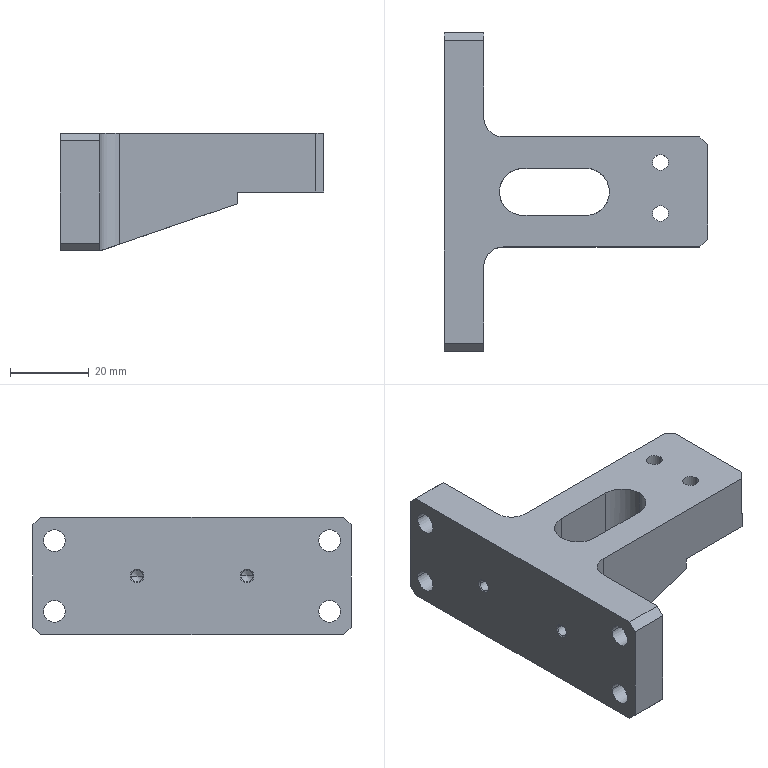Component | SolidWorks | AX.B92.SA.7371.20-2 | 1 solid | 60 faces | box 67 x 81 x 30 mm | volume 48369 mm3 | cylinder 25 | plane 23 | cone 12 | commonest cylinder face diameters 5.5 x8 4 x4 6 x4 3 x4 12 x3 10 x2 | material 6061
build123d program:
from build123d import *

# Parameters (mm, degrees)
BOSS_EXTRUDE1_DEPTH                 = 15
SKETCH2_W                           = 28
SKETCH2_H                           = 22
CUT_EXTRUDE1_DEPTH                  = 15
SKETCH3_W                           = 81
SKETCH3_H                           = 30
BOSS_EXTRUDE2_DEPTH                 = 10
FILLET2_R                           = 5
CHAMFER1_SIZE                       = 2
CUT_EXTRUDE2_DEPTH                  = 84.841
CUT_EXTRUDE3_DEPTH                  = 50
F_5_5_5_5_DIAMETER_HOLE1_D          = 5.5
SIZE_MM_DOWEL_PIN_HOLE1_D           = 3
SIZE_MM_DOWEL_PIN_HOLE1_DEPTH       = 10
SIZE_MM_DOWEL_PIN_HOLE1_CSINK_D     = 3.5
SIZE_MM_DOWEL_PIN_HOLE1_CSINK_ANGLE = 90
SIZE_MM_DOWEL_PIN_HOLE1_TIP         = 0.9013
SKETCH10_R                          = 3
CUT_EXTRUDE4_DEPTH                  = 4
M4_TAPPED_HOLE1_D                   = 4
M4_TAPPED_HOLE1_CSINK_D             = 4.05
M4_TAPPED_HOLE1_CSINK_ANGLE         = 90


with BuildPart() as part:
    # Sketch1 → Boss-Extrude1 (new, symmetric)
    with BuildSketch(Plane(origin=(0, 0, 0), x_dir=(1, 0, 0), z_dir=(0, 1, 0))):
        Polygon((0, 0), (-14, 0), (-14, 57), (14, 57), (14, 0), align=None)
    extrude(amount=BOSS_EXTRUDE1_DEPTH, both=True)

    # Sketch2 → Cut-Extrude1 (cut)
    with BuildSketch(Plane(origin=(0, 15, 0), x_dir=(1, 0, 0), z_dir=(0, 1, 0))):
        with Locations((0, 11)):
            Rectangle(SKETCH2_W, SKETCH2_H)
    extrude(amount=-CUT_EXTRUDE1_DEPTH, mode=Mode.SUBTRACT)

    # Sketch3 → Boss-Extrude2 (add)
    with BuildSketch(Plane(origin=(0, 0, -57), x_dir=(-1, 0, 0), z_dir=(0, 0, -1))):
        Rectangle(SKETCH3_W, SKETCH3_H)
    extrude(amount=BOSS_EXTRUDE2_DEPTH)

    # Fillet2
    fillet2_edges = [part.edges().sort_by_distance(p)[0] for p in [
        (-14, 0, -57),
        (14, 0, -57),
    ]]
    fillet(fillet2_edges, radius=FILLET2_R)

    # Chamfer1
    chamfer1_edges = [part.edges().sort_by_distance(p)[0] for p in [
        (14, -7.5, 0),
        (-14, -7.5, 0),
        (40.5, 15, -62),
        (40.5, -15, -62),
        (-40.5, -15, -62),
        (-40.5, 15, -62),
    ]]
    chamfer(chamfer1_edges, length=CHAMFER1_SIZE)

    # Sketch4 → Cut-Extrude2 (cut, through all)
    with BuildSketch(Plane(origin=(0, 15, 0), x_dir=(1, 0, 0), z_dir=(0, 1, 0))):
        with BuildLine():
            Line((6, 47), (6, 31))
            ThreePointArc((6, 31), (0, 25), (-6, 31))
            Line((-6, 31), (-6, 47))
            ThreePointArc((-6, 47), (0, 53), (6, 47))
        make_face()
    extrude(amount=-CUT_EXTRUDE2_DEPTH, mode=Mode.SUBTRACT)

    # Sketch5 → Cut-Extrude3 (cut, symmetric)
    with BuildSketch(Plane.ZY.offset(14)):
        Polygon((-22, 3), (-57, 15), (-22, 15), align=None)
    extrude(amount=CUT_EXTRUDE3_DEPTH, both=True, mode=Mode.SUBTRACT)

    # 5.5 _5.5_ Diameter Hole1 (through all)
    with Locations(Plane.XY.offset(-57)):
        with Locations((-35, 9), (-35, -9), (35, -9), (35, 9)):
            Hole(F_5_5_5_5_DIAMETER_HOLE1_D / 2)

    # Size mm Dowel Pin Hole1
    with Locations(Plane(origin=(0, 0, -67), x_dir=(-1, 0, 0), z_dir=(0, 0, -1))):
        with Locations((-14, 0), (14, 0)):
            CounterSinkHole(SIZE_MM_DOWEL_PIN_HOLE1_D / 2, SIZE_MM_DOWEL_PIN_HOLE1_CSINK_D / 2, depth=SIZE_MM_DOWEL_PIN_HOLE1_DEPTH, counter_sink_angle=SIZE_MM_DOWEL_PIN_HOLE1_CSINK_ANGLE)
            with Locations((0, 0, -(SIZE_MM_DOWEL_PIN_HOLE1_DEPTH + SIZE_MM_DOWEL_PIN_HOLE1_TIP / 2))):  # 118° drill point
                Cone(0, SIZE_MM_DOWEL_PIN_HOLE1_D / 2, SIZE_MM_DOWEL_PIN_HOLE1_TIP, mode=Mode.SUBTRACT)

    # Sketch10 → Cut-Extrude4 (cut)
    with BuildSketch(Plane(origin=(0, 0, 0), x_dir=(1, 0, 0), z_dir=(0, 1, 0))):
        with Locations(Location((-7.5, 12, 0), (0, 0, 270))):
            Circle(SKETCH10_R)
        with Locations(Location((5.5, 12, 0), (0, 0, 270))):
            Circle(SKETCH10_R)
    extrude(amount=-CUT_EXTRUDE4_DEPTH, mode=Mode.SUBTRACT)

    # M4 Tapped Hole1 (through all)
    with Locations(Plane(origin=(0, -4, 0), x_dir=(1, 0, 0), z_dir=(0, 1, 0))):
        with Locations((-7.5, 12), (5.5, 12)):
            CounterSinkHole(M4_TAPPED_HOLE1_D / 2, M4_TAPPED_HOLE1_CSINK_D / 2, counter_sink_angle=M4_TAPPED_HOLE1_CSINK_ANGLE)


solid = part.part

# Placed as in the assembly
solid = solid.moved(Location((209.421, 53.688, 57.972), (-90, 90, 0)))